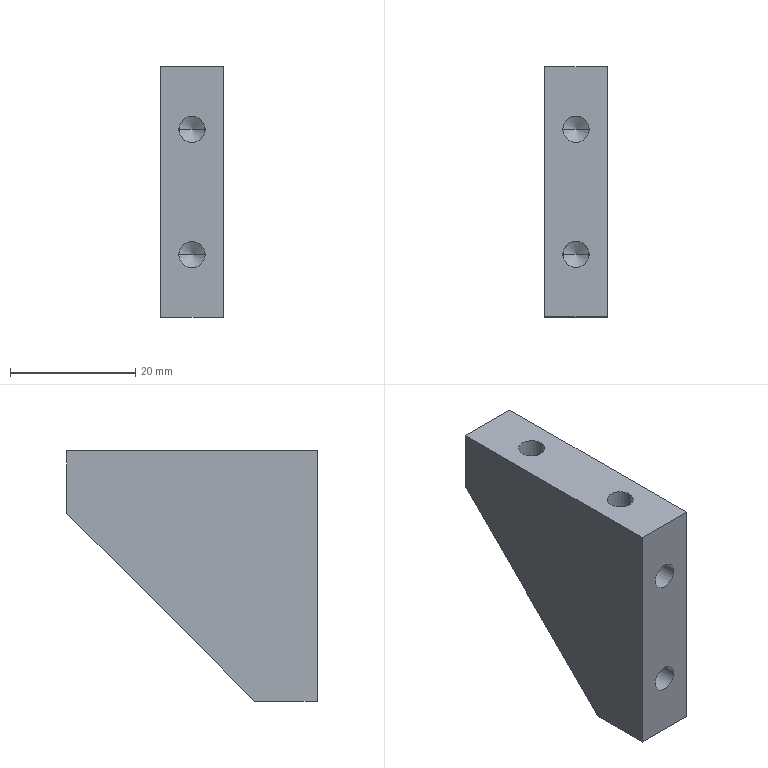Component | SolidWorks | 022-1 | 1 solid | 27 faces | box 10 x 40 x 40 mm | volume 10839 mm3 | cylinder 12 | cone 8 | plane 7 | commonest cylinder face diameters 4.2 x12 | material AL6061
build123d program:
from build123d import *

# Parameters (mm, degrees)
SKETCH1_W             = 40
SKETCH1_H             = 40
BOSS_EXTRUDE1_DEPTH   = 10
CUT_EXTRUDE1_DEPTH    = 31
M5_TAPPED_HOLE1_D     = 4.2
M5_TAPPED_HOLE1_DEPTH = 12.4
M5_TAPPED_HOLE1_TIP   = 1.262
M5_TAPPED_HOLE2_D     = 4.2
M5_TAPPED_HOLE2_DEPTH = 12.4
M5_TAPPED_HOLE2_TIP   = 1.262


with BuildPart() as part:
    # Sketch1 → Boss-Extrude1 (new body)
    with BuildSketch(Plane.XY):
        Rectangle(SKETCH1_W, SKETCH1_H)
    extrude(amount=BOSS_EXTRUDE1_DEPTH)

    # Sketch2 → Cut-Extrude1 (cut, through all)
    with BuildSketch(Plane.XY.offset(10)):
        Polygon((-10, 20), (20, -10), (20, 20), align=None)
    extrude(amount=-CUT_EXTRUDE1_DEPTH, mode=Mode.SUBTRACT)

    # M5 Tapped Hole1
    with Locations(Plane.ZY.offset(20)):
        with Locations((5, -10), (5, 10)):
            Hole(M5_TAPPED_HOLE1_D / 2, depth=M5_TAPPED_HOLE1_DEPTH)
            with Locations((0, 0, -(M5_TAPPED_HOLE1_DEPTH + M5_TAPPED_HOLE1_TIP / 2))):  # 118° drill point
                Cone(0, M5_TAPPED_HOLE1_D / 2, M5_TAPPED_HOLE1_TIP, mode=Mode.SUBTRACT)

    # M5 Tapped Hole2
    with Locations(Plane(origin=(0, -20, 0), x_dir=(-1, 0, 0), z_dir=(0, -1, 0))):
        with Locations((10, -5), (-10, -5)):
            Hole(M5_TAPPED_HOLE2_D / 2, depth=M5_TAPPED_HOLE2_DEPTH)
            with Locations((0, 0, -(M5_TAPPED_HOLE2_DEPTH + M5_TAPPED_HOLE2_TIP / 2))):  # 118° drill point
                Cone(0, M5_TAPPED_HOLE2_D / 2, M5_TAPPED_HOLE2_TIP, mode=Mode.SUBTRACT)


solid = part.part

# Placed as in the assembly
solid = solid.moved(Location((-245.455, -85.942, -159.304), (0, 90, 0)))